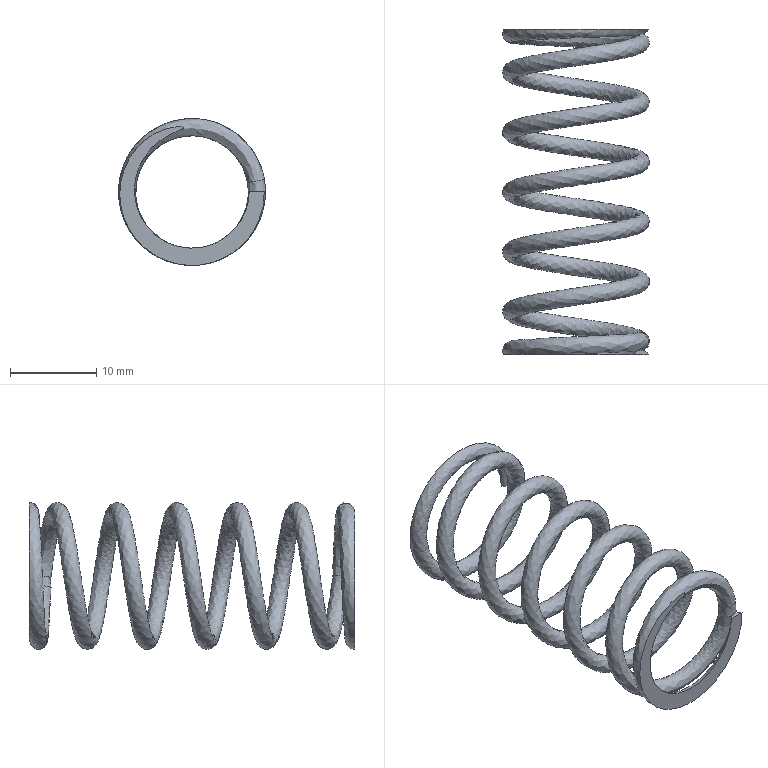Component | NX | VALVE_BODY_SPRING | 1 solid | 9 faces | volume 961 mm3 | spline 5 | plane 4